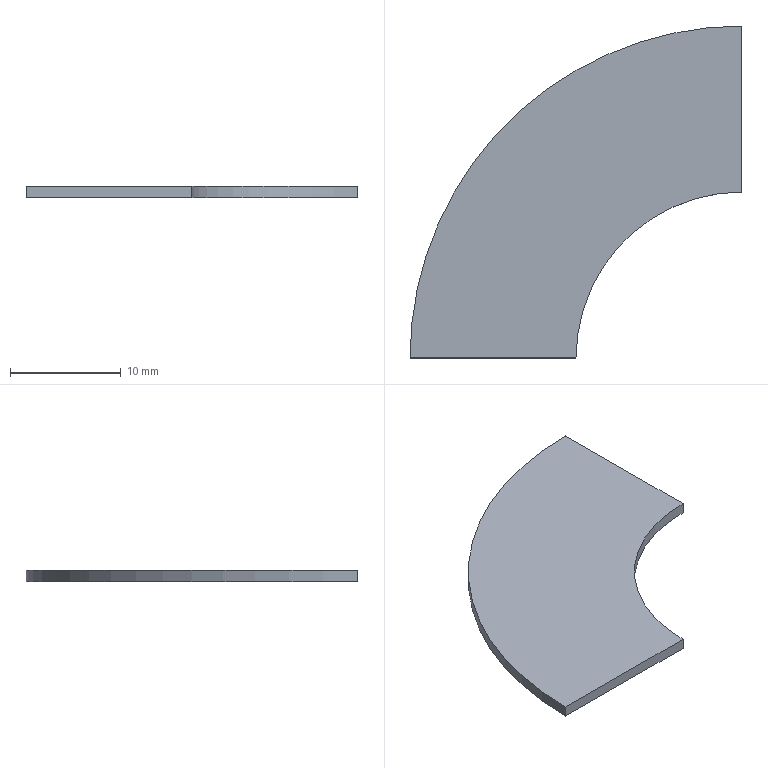Component | SolidWorks | Mirror_w4-2 | 1 solid | 6 faces | box 30 x 30 x 1 mm | volume 530 mm3 | plane 4 | cylinder 2 | commonest cylinder face diameters 30 x1 60 x1
STEP:
#1=COLOUR_RGB('',0.7922,0.8196,0.9333);
#2=FILL_AREA_STYLE_COLOUR('',#1);
#3=FILL_AREA_STYLE('',(#2));
#4=SURFACE_STYLE_FILL_AREA(#3);
#5=SURFACE_SIDE_STYLE('',(#4));
#6=SURFACE_STYLE_USAGE(.BOTH.,#5);
#7=PRESENTATION_STYLE_ASSIGNMENT((#6));
#8=CARTESIAN_POINT('',(-9.252,28.376,-1.28));
#9=VERTEX_POINT('',#8);
#10=CARTESIAN_POINT('',(-8.661,28.967,-1.28));
#11=VERTEX_POINT('',#10);
#12=CARTESIAN_POINT('',(-8.661,28.376,-1.28));
#13=DIRECTION('',(0.,-0.,-1.));
#14=DIRECTION('',(0.,1.,0.));
#15=AXIS2_PLACEMENT_3D('',#12,#13,#14);
#16=CIRCLE('',#15,0.5906);
#17=EDGE_CURVE('',#9,#11,#16,.T.);
#18=ORIENTED_EDGE('',*,*,#17,.F.);
#19=CARTESIAN_POINT('',(-9.252,28.376,-1.319));
#20=VERTEX_POINT('',#19);
#21=CARTESIAN_POINT('',(-9.252,28.376,-1.319));
#22=DIRECTION('',(-0.,0.,1.));
#23=VECTOR('',#22,39.37);
#24=LINE('',#21,#23);
#25=EDGE_CURVE('',#20,#9,#24,.T.);
#26=ORIENTED_EDGE('',*,*,#25,.F.);
#27=CARTESIAN_POINT('',(-8.661,28.967,-1.319));
#28=VERTEX_POINT('',#27);
#29=CARTESIAN_POINT('',(-8.661,28.376,-1.319));
#30=DIRECTION('',(0.,-0.,-1.));
#31=DIRECTION('',(0.,1.,0.));
#32=AXIS2_PLACEMENT_3D('',#29,#30,#31);
#33=CIRCLE('',#32,0.5906);
#34=EDGE_CURVE('',#20,#28,#33,.T.);
#35=ORIENTED_EDGE('',*,*,#34,.T.);
#36=CARTESIAN_POINT('',(-8.661,28.967,-1.319));
#37=DIRECTION('',(-0.,0.,1.));
#38=VECTOR('',#37,39.37);
#39=LINE('',#36,#38);
#40=EDGE_CURVE('',#28,#11,#39,.T.);
#41=ORIENTED_EDGE('',*,*,#40,.T.);
#42=EDGE_LOOP('',(#18,#26,#35,#41));
#43=FACE_OUTER_BOUND('',#42,.T.);
#44=CARTESIAN_POINT('',(-8.661,28.376,-1.319));
#45=DIRECTION('',(-0.,0.,1.));
#46=DIRECTION('',(0.,-1.,0.));
#47=AXIS2_PLACEMENT_3D('',#44,#45,#46);
#48=CYLINDRICAL_SURFACE('',#47,0.5906);
#49=ADVANCED_FACE('',(#43),#48,.F.);
#50=CARTESIAN_POINT('',(-8.661,29.557,-1.28));
#51=VERTEX_POINT('',#50);
#52=CARTESIAN_POINT('',(-8.661,28.967,-1.28));
#53=DIRECTION('',(0.,1.,0.));
#54=VECTOR('',#53,39.37);
#55=LINE('',#52,#54);
#56=EDGE_CURVE('',#11,#51,#55,.T.);
#57=ORIENTED_EDGE('',*,*,#56,.F.);
#58=ORIENTED_EDGE('',*,*,#40,.F.);
#59=CARTESIAN_POINT('',(-8.661,29.557,-1.319));
#60=VERTEX_POINT('',#59);
#61=CARTESIAN_POINT('',(-8.661,28.967,-1.319));
#62=DIRECTION('',(0.,1.,0.));
#63=VECTOR('',#62,39.37);
#64=LINE('',#61,#63);
#65=EDGE_CURVE('',#28,#60,#64,.T.);
#66=ORIENTED_EDGE('',*,*,#65,.T.);
#67=CARTESIAN_POINT('',(-8.661,29.557,-1.319));
#68=DIRECTION('',(-0.,0.,1.));
#69=VECTOR('',#68,39.37);
#70=LINE('',#67,#69);
#71=EDGE_CURVE('',#60,#51,#70,.T.);
#72=ORIENTED_EDGE('',*,*,#71,.T.);
#73=EDGE_LOOP('',(#57,#58,#66,#72));
#74=FACE_OUTER_BOUND('',#73,.T.);
#75=CARTESIAN_POINT('',(-8.661,28.967,-1.319));
#76=DIRECTION('',(-1.,0.,-0.));
#77=DIRECTION('',(0.,-0.,-1.));
#78=AXIS2_PLACEMENT_3D('',#75,#76,#77);
#79=PLANE('',#78);
#80=ADVANCED_FACE('',(#74),#79,.F.);
#81=CARTESIAN_POINT('',(-9.843,28.376,-1.28));
#82=VERTEX_POINT('',#81);
#83=CARTESIAN_POINT('',(-8.661,28.376,-1.28));
#84=DIRECTION('',(-0.,0.,1.));
#85=DIRECTION('',(0.,1.,0.));
#86=AXIS2_PLACEMENT_3D('',#83,#84,#85);
#87=CIRCLE('',#86,1.181);
#88=EDGE_CURVE('',#51,#82,#87,.T.);
#89=ORIENTED_EDGE('',*,*,#88,.F.);
#90=ORIENTED_EDGE('',*,*,#71,.F.);
#91=CARTESIAN_POINT('',(-9.843,28.376,-1.319));
#92=VERTEX_POINT('',#91);
#93=CARTESIAN_POINT('',(-8.661,28.376,-1.319));
#94=DIRECTION('',(-0.,0.,1.));
#95=DIRECTION('',(0.,1.,0.));
#96=AXIS2_PLACEMENT_3D('',#93,#94,#95);
#97=CIRCLE('',#96,1.181);
#98=EDGE_CURVE('',#60,#92,#97,.T.);
#99=ORIENTED_EDGE('',*,*,#98,.T.);
#100=CARTESIAN_POINT('',(-9.843,28.376,-1.319));
#101=DIRECTION('',(-0.,0.,1.));
#102=VECTOR('',#101,39.37);
#103=LINE('',#100,#102);
#104=EDGE_CURVE('',#92,#82,#103,.T.);
#105=ORIENTED_EDGE('',*,*,#104,.T.);
#106=EDGE_LOOP('',(#89,#90,#99,#105));
#107=FACE_OUTER_BOUND('',#106,.T.);
#108=CARTESIAN_POINT('',(-8.661,28.376,-1.319));
#109=DIRECTION('',(-0.,0.,1.));
#110=DIRECTION('',(0.,-1.,0.));
#111=AXIS2_PLACEMENT_3D('',#108,#109,#110);
#112=CYLINDRICAL_SURFACE('',#111,1.181);
#113=ADVANCED_FACE('',(#107),#112,.T.);
#114=CARTESIAN_POINT('',(-9.252,28.376,-1.28));
#115=DIRECTION('',(1.,-0.,0.));
#116=VECTOR('',#115,39.37);
#117=LINE('',#114,#116);
#118=EDGE_CURVE('',#82,#9,#117,.T.);
#119=ORIENTED_EDGE('',*,*,#118,.F.);
#120=ORIENTED_EDGE('',*,*,#104,.F.);
#121=CARTESIAN_POINT('',(-9.252,28.376,-1.319));
#122=DIRECTION('',(1.,-0.,0.));
#123=VECTOR('',#122,39.37);
#124=LINE('',#121,#123);
#125=EDGE_CURVE('',#92,#20,#124,.T.);
#126=ORIENTED_EDGE('',*,*,#125,.T.);
#127=ORIENTED_EDGE('',*,*,#25,.T.);
#128=EDGE_LOOP('',(#119,#120,#126,#127));
#129=FACE_OUTER_BOUND('',#128,.T.);
#130=CARTESIAN_POINT('',(-9.252,28.376,-1.319));
#131=DIRECTION('',(0.,1.,0.));
#132=DIRECTION('',(-0.,0.,1.));
#133=AXIS2_PLACEMENT_3D('',#130,#131,#132);
#134=PLANE('',#133);
#135=ADVANCED_FACE('',(#129),#134,.F.);
#136=ORIENTED_EDGE('',*,*,#34,.F.);
#137=ORIENTED_EDGE('',*,*,#125,.F.);
#138=ORIENTED_EDGE('',*,*,#98,.F.);
#139=ORIENTED_EDGE('',*,*,#65,.F.);
#140=EDGE_LOOP('',(#136,#137,#138,#139));
#141=FACE_OUTER_BOUND('',#140,.T.);
#142=CARTESIAN_POINT('',(-8.661,28.376,-1.319));
#143=DIRECTION('',(0.,-0.,-1.));
#144=DIRECTION('',(0.,1.,0.));
#145=AXIS2_PLACEMENT_3D('',#142,#143,#144);
#146=PLANE('',#145);
#147=ADVANCED_FACE('',(#141),#146,.T.);
#148=ORIENTED_EDGE('',*,*,#17,.T.);
#149=ORIENTED_EDGE('',*,*,#56,.T.);
#150=ORIENTED_EDGE('',*,*,#88,.T.);
#151=ORIENTED_EDGE('',*,*,#118,.T.);
#152=EDGE_LOOP('',(#148,#149,#150,#151));
#153=FACE_OUTER_BOUND('',#152,.T.);
#154=CARTESIAN_POINT('',(-8.661,28.376,-1.28));
#155=DIRECTION('',(0.,-0.,-1.));
#156=DIRECTION('',(0.,1.,0.));
#157=AXIS2_PLACEMENT_3D('',#154,#155,#156);
#158=PLANE('',#157);
#159=ADVANCED_FACE('',(#153),#158,.F.);
#160=CLOSED_SHELL('',(#49,#80,#113,#135,#147,#159));
#161=MANIFOLD_SOLID_BREP('',#160);
#162=STYLED_ITEM('',(#7),#161);
#163=PRESENTATION_LAYER_ASSIGNMENT('','',(#162));
#164=(LENGTH_UNIT()NAMED_UNIT(*)SI_UNIT($,.METRE.));
#165=LENGTH_MEASURE_WITH_UNIT(LENGTH_MEASURE(0.0254),#164);
#166=DIMENSIONAL_EXPONENTS(1.,0.,0.,0.,0.,0.,0.);
#167=(CONVERSION_BASED_UNIT('',#165)LENGTH_UNIT()NAMED_UNIT(#166));
#168=UNCERTAINTY_MEASURE_WITH_UNIT(LENGTH_MEASURE(0.00001),#167,'','');
#169=(NAMED_UNIT(*)PLANE_ANGLE_UNIT()SI_UNIT($,.RADIAN.));
#170=(NAMED_UNIT(*)SI_UNIT($,.STERADIAN.)SOLID_ANGLE_UNIT());
#171=(GEOMETRIC_REPRESENTATION_CONTEXT(3)GLOBAL_UNCERTAINTY_ASSIGNED_CONTEXT((#168))GLOBAL_UNIT_ASSIGNED_CONTEXT((#167,#169,#170))REPRESENTATION_CONTEXT('',''));
#172=MECHANICAL_DESIGN_GEOMETRIC_PRESENTATION_REPRESENTATION('',(#162),#171);
#173=CARTESIAN_POINT('',(0.,0.,0.));
#174=DIRECTION('',(0.,0.,1.));
#175=DIRECTION('',(1.,0.,0.));
#176=AXIS2_PLACEMENT_3D('',#173,#174,#175);
#177=(LENGTH_UNIT()NAMED_UNIT(*)SI_UNIT($,.METRE.));
#178=LENGTH_MEASURE_WITH_UNIT(LENGTH_MEASURE(0.0254),#177);
#179=DIMENSIONAL_EXPONENTS(1.,0.,0.,0.,0.,0.,0.);
#180=(CONVERSION_BASED_UNIT('',#178)LENGTH_UNIT()NAMED_UNIT(#179));
#181=UNCERTAINTY_MEASURE_WITH_UNIT(LENGTH_MEASURE(0.00001),#180,'','');
#182=(NAMED_UNIT(*)PLANE_ANGLE_UNIT()SI_UNIT($,.RADIAN.));
#183=(NAMED_UNIT(*)SI_UNIT($,.STERADIAN.)SOLID_ANGLE_UNIT());
#184=(GEOMETRIC_REPRESENTATION_CONTEXT(3)GLOBAL_UNCERTAINTY_ASSIGNED_CONTEXT((#181))GLOBAL_UNIT_ASSIGNED_CONTEXT((#180,#182,#183))REPRESENTATION_CONTEXT('',''));
#185=ADVANCED_BREP_SHAPE_REPRESENTATION('',(#161,#176),#184);